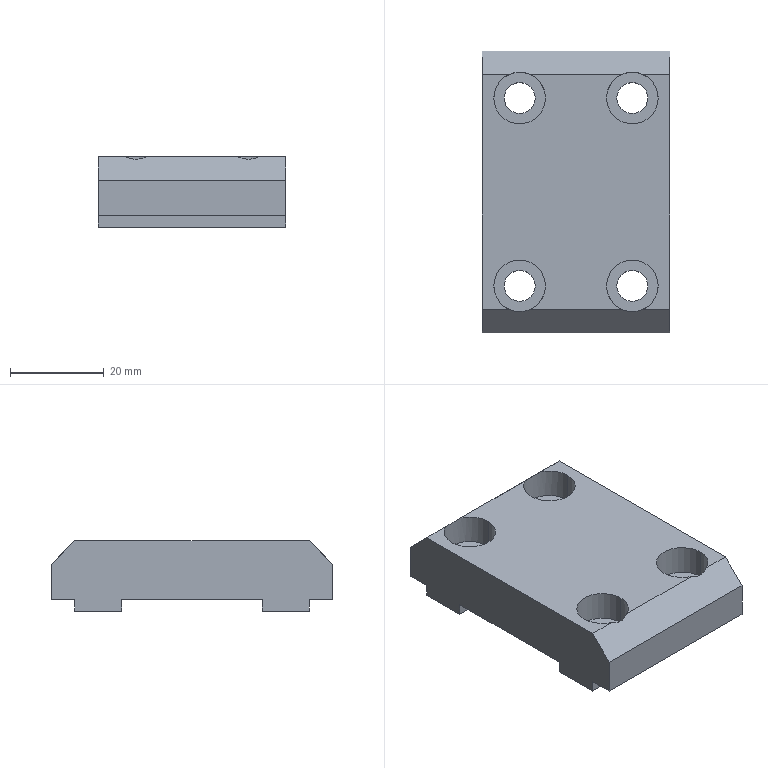Component | SolidWorks | Q1-A12-S21-Q1D.SLDASQ-1_Q1-A12-S21-Q1D-01A-1 | 1 solid | 40 faces | volume 26668 mm3 | plane 20 | cylinder 18 | cone 2 | commonest cylinder face diameters 11 x8 6.6 x8 6 x2 | material Q235-Steel